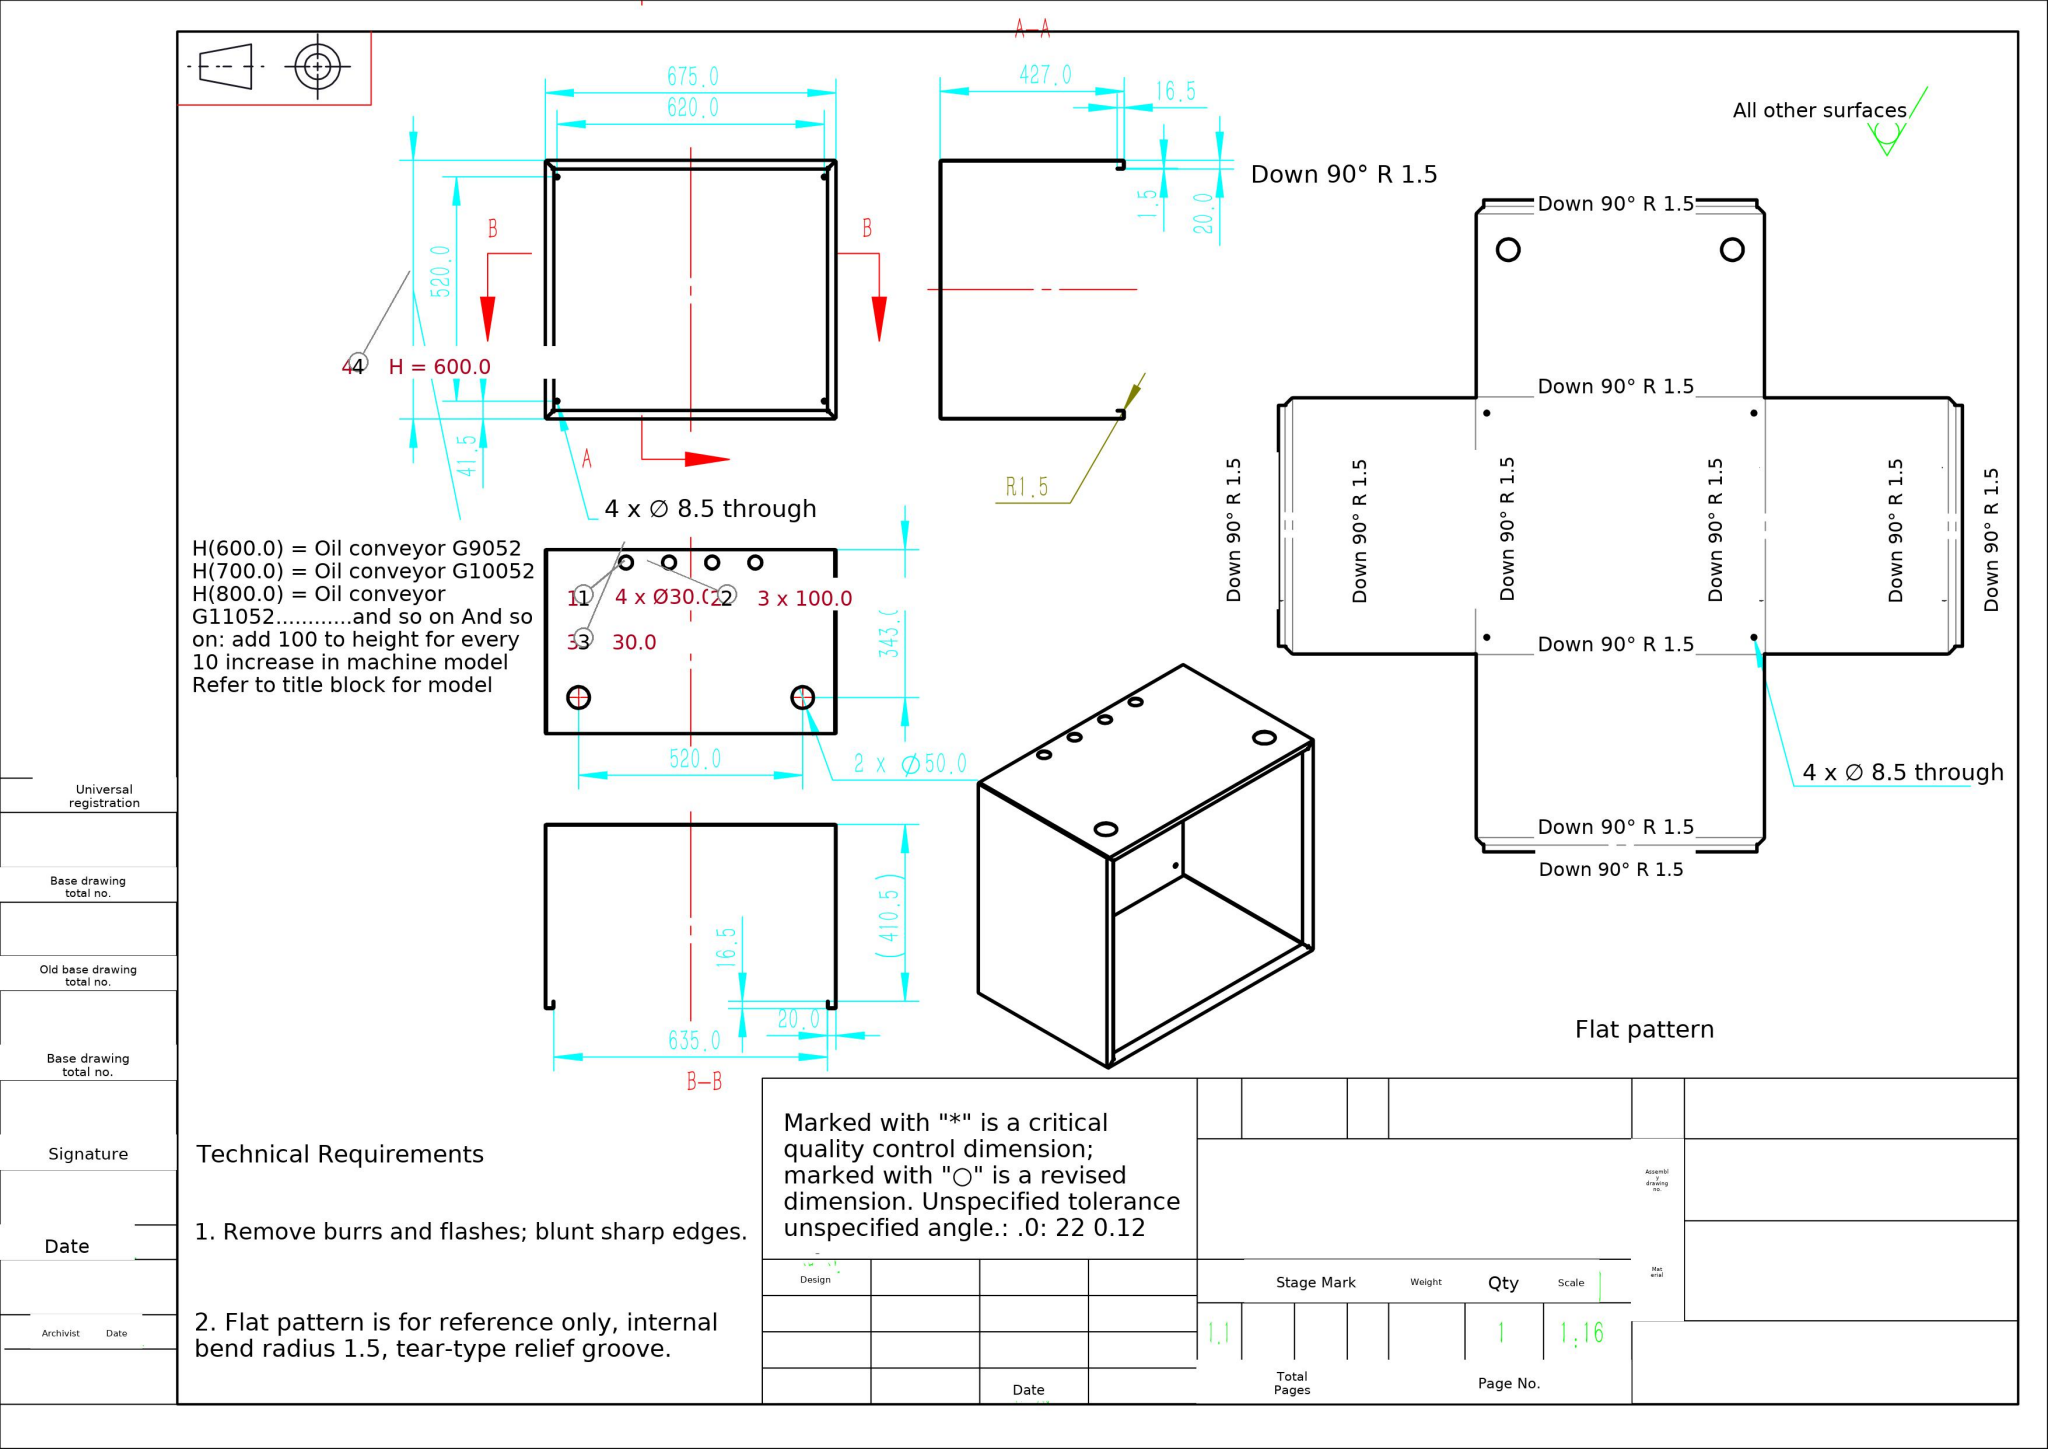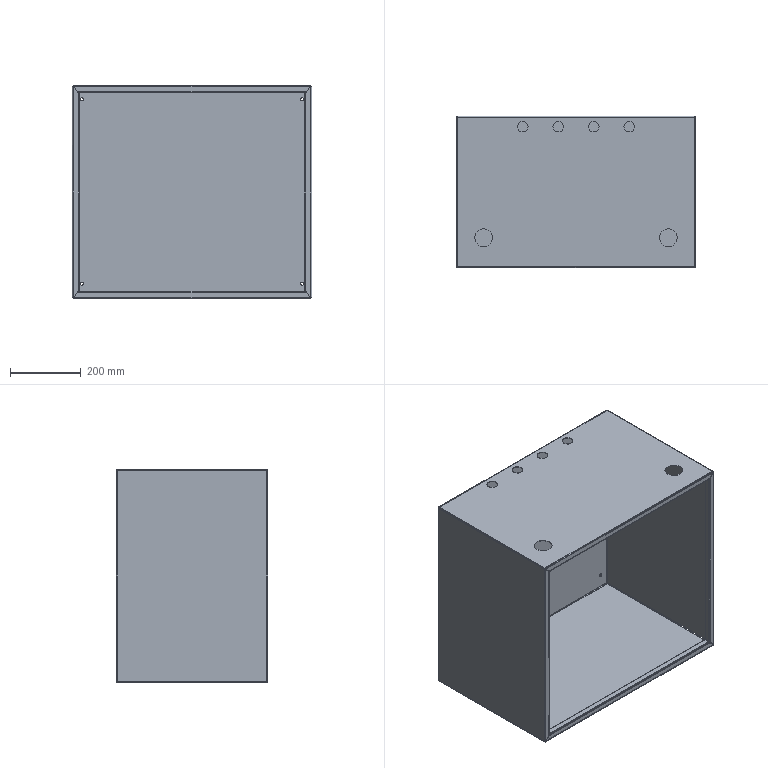Part | SolidWorks | mm | 1 solid | 162 faces | box 675 x 427 x 600 mm | volume 2320676 mm3 | plane 110 | cylinder 44 | spline 8 | commonest cylinder face diameters 6 x12 3 x12 8.5 x8 30 x8 50 x4